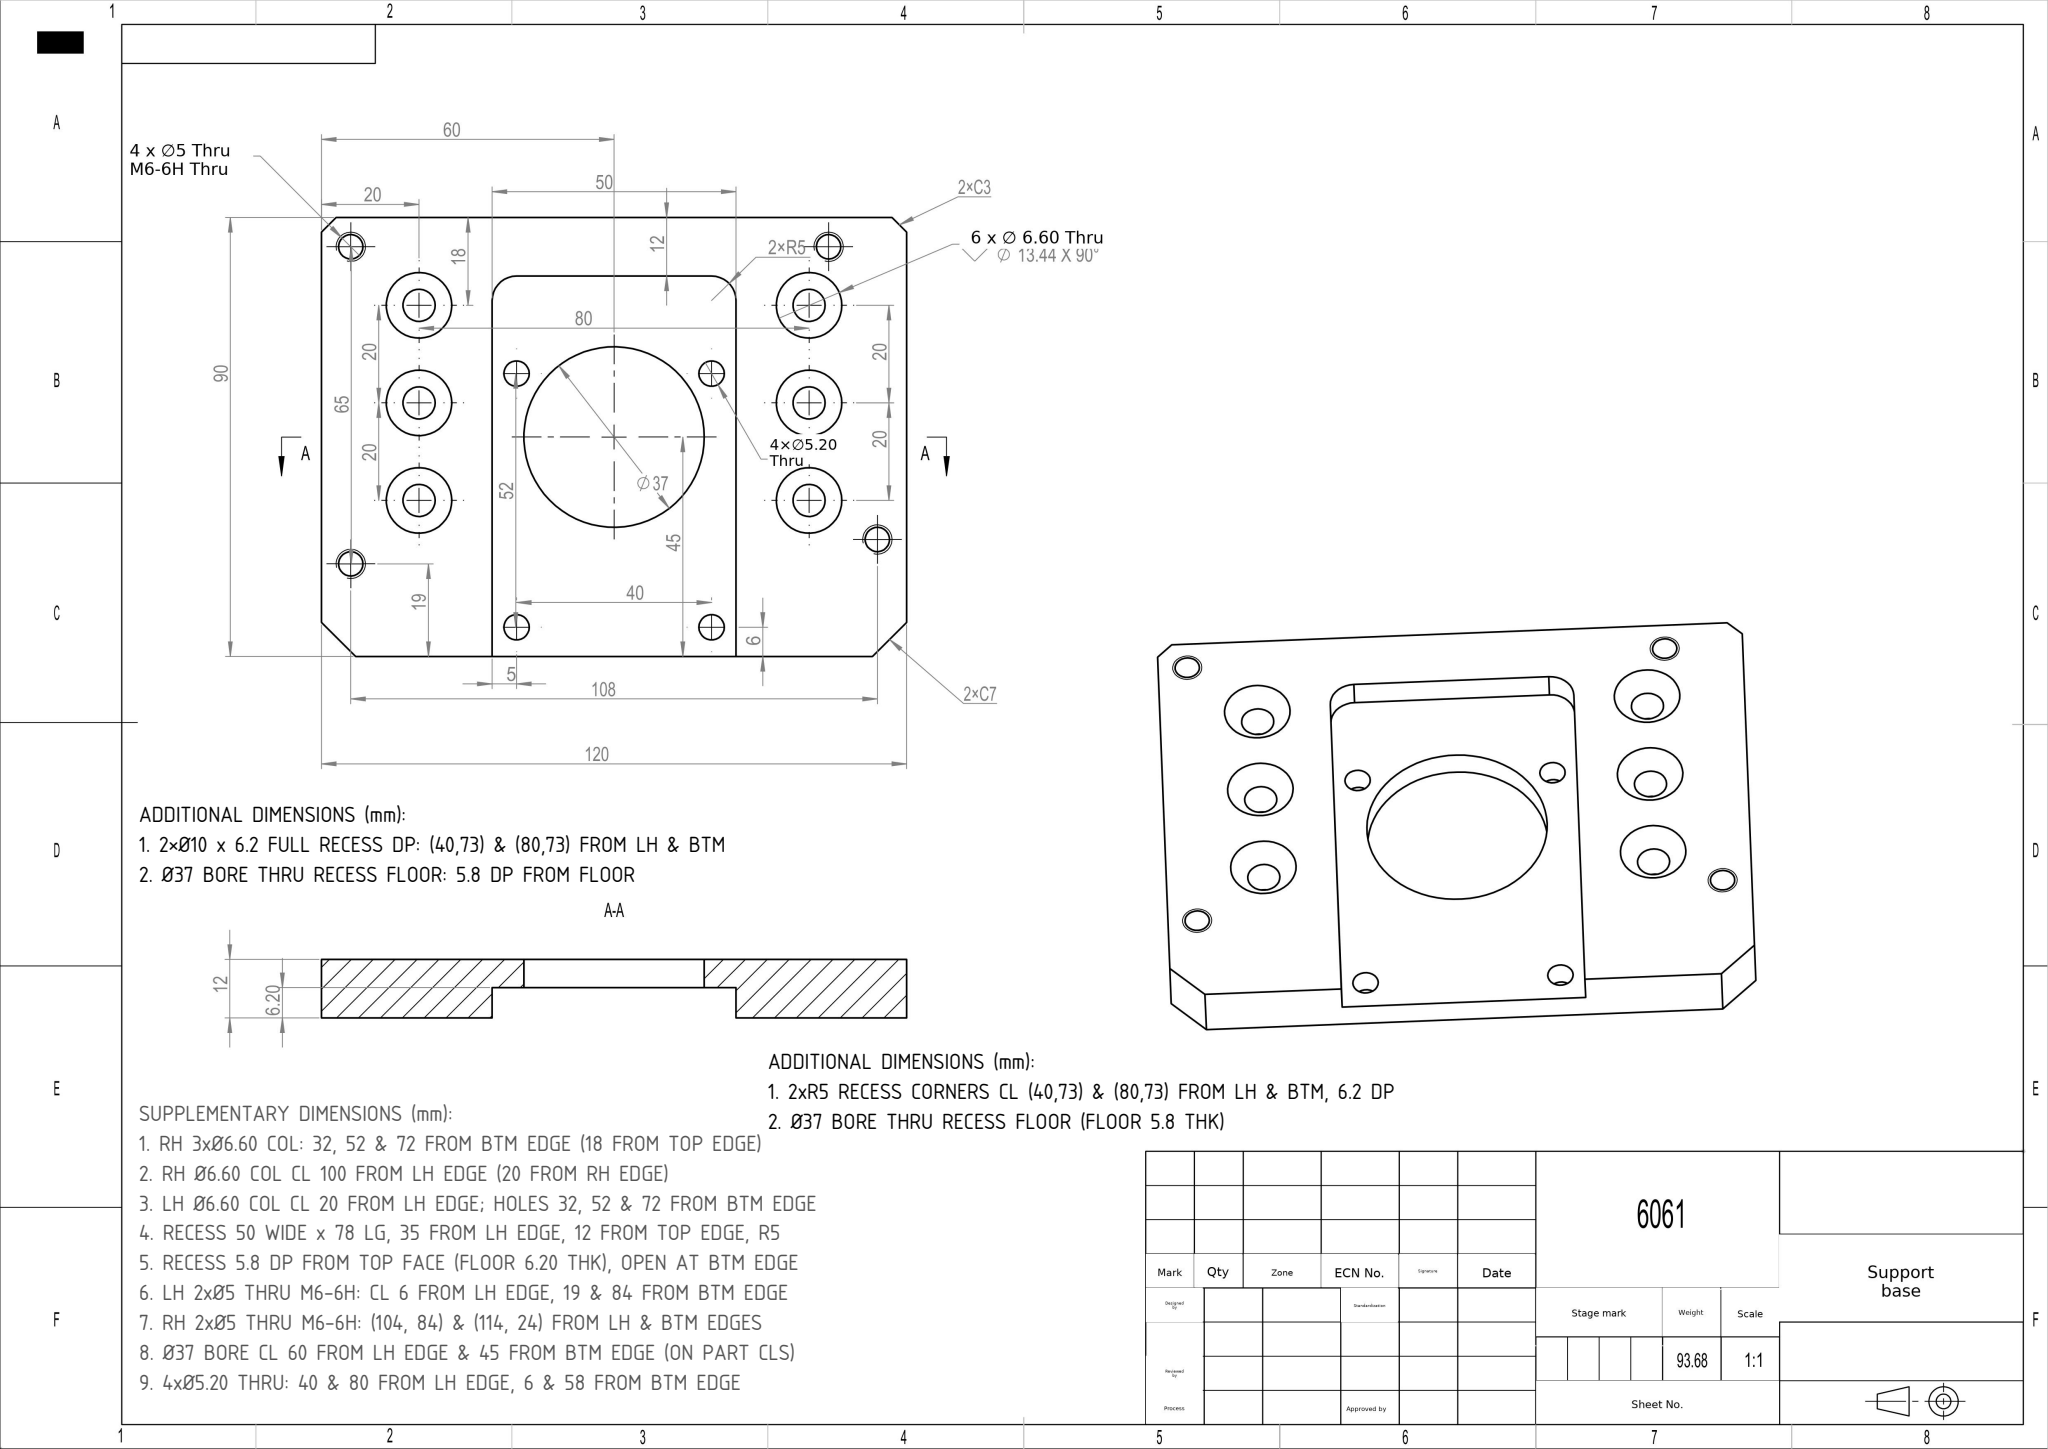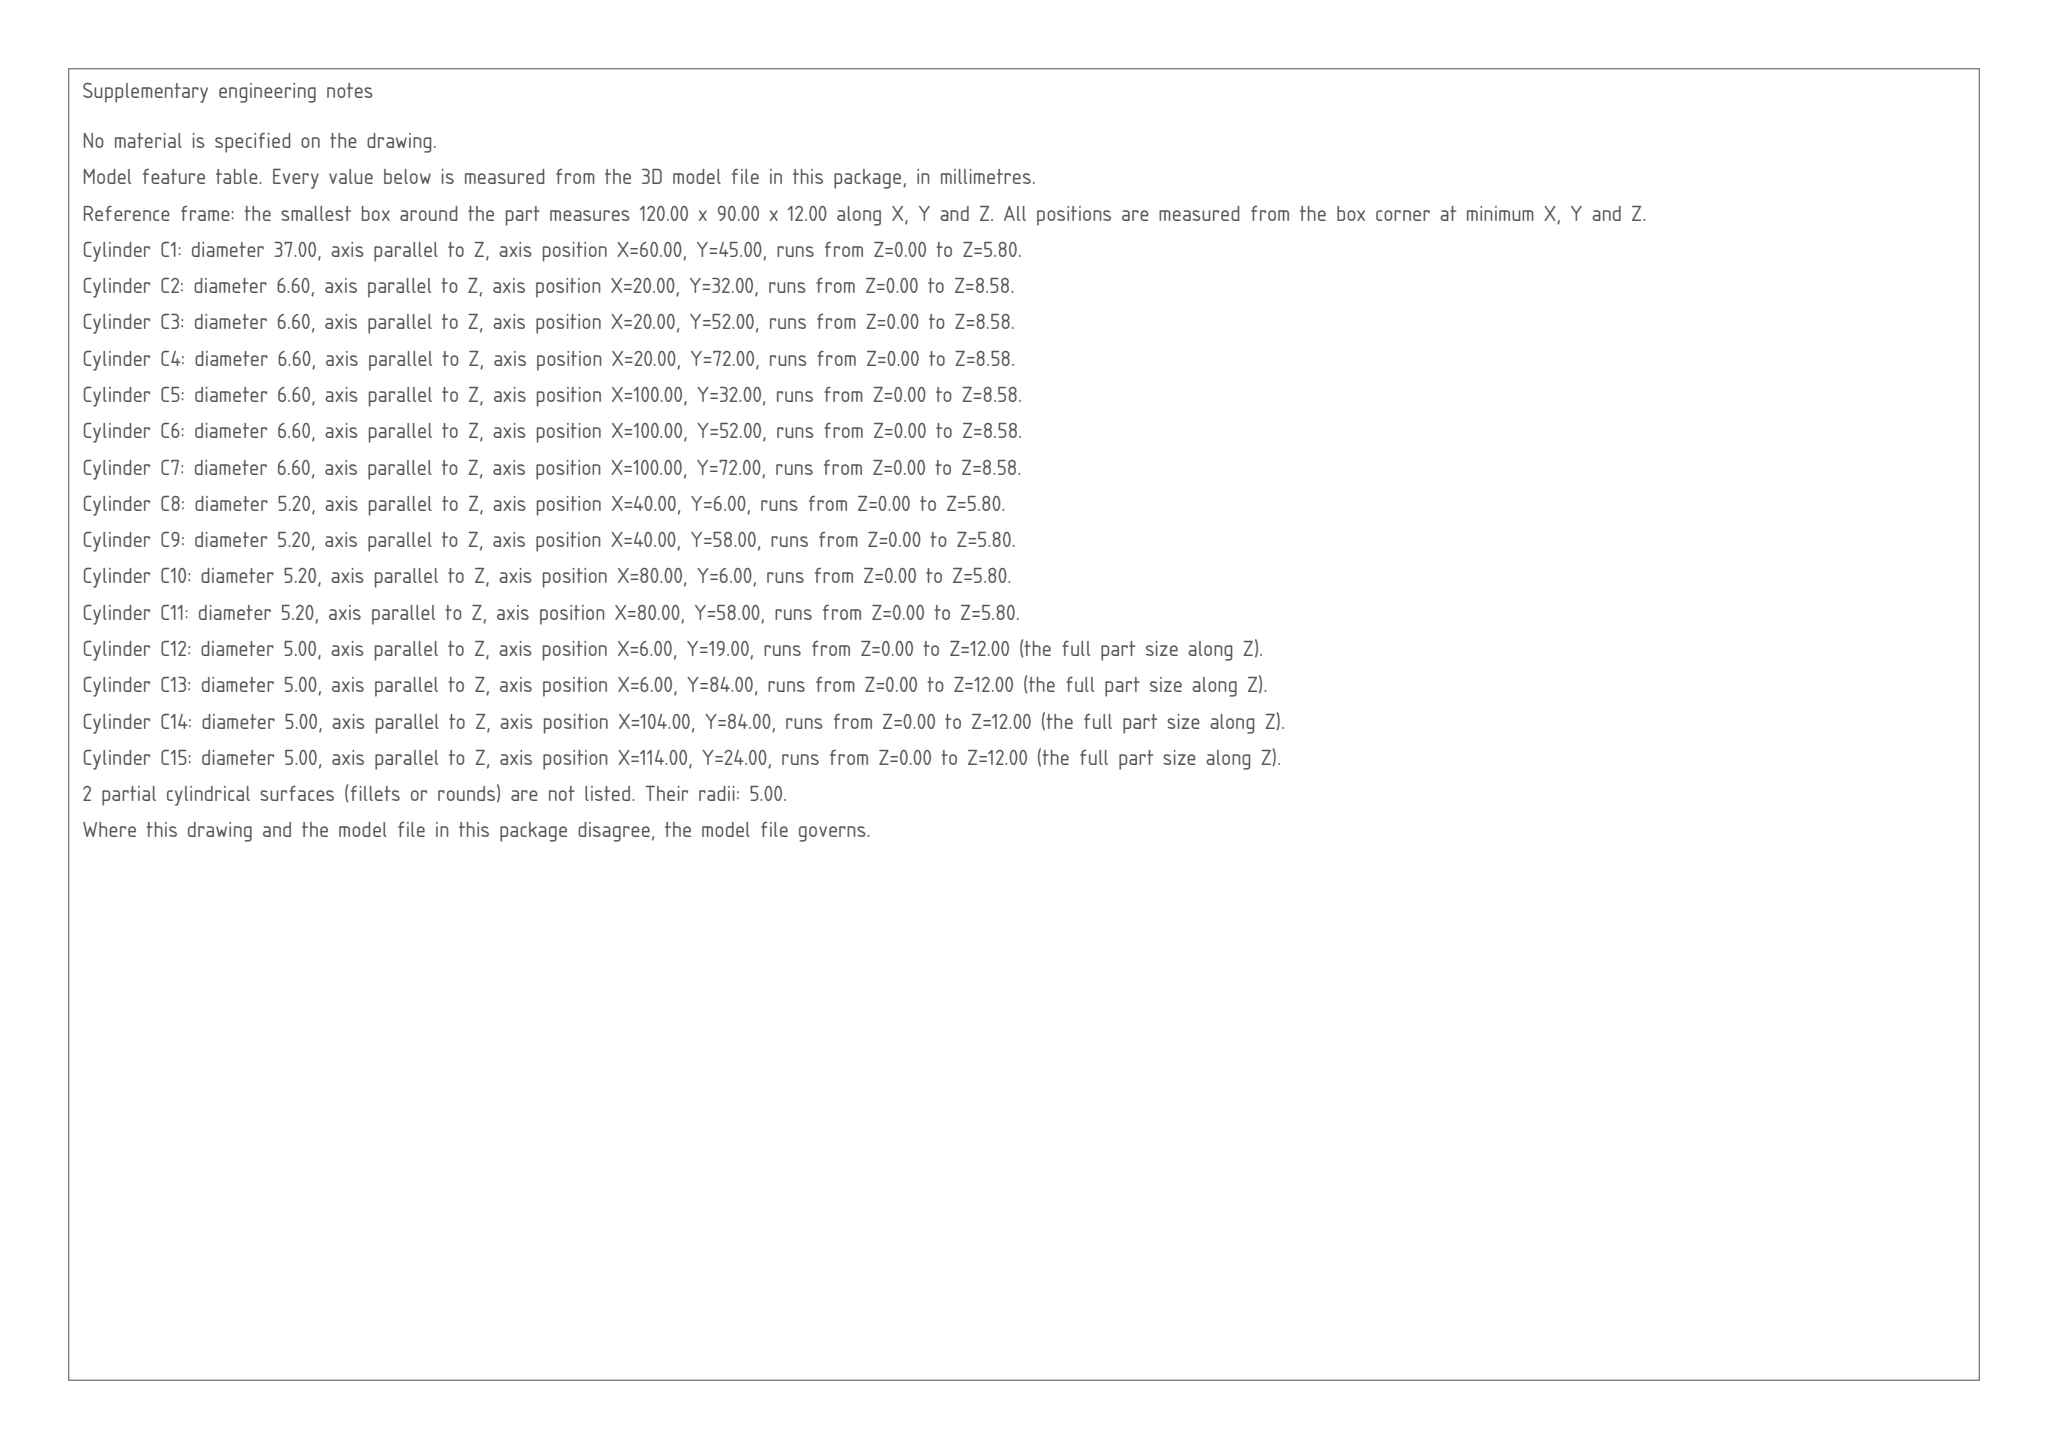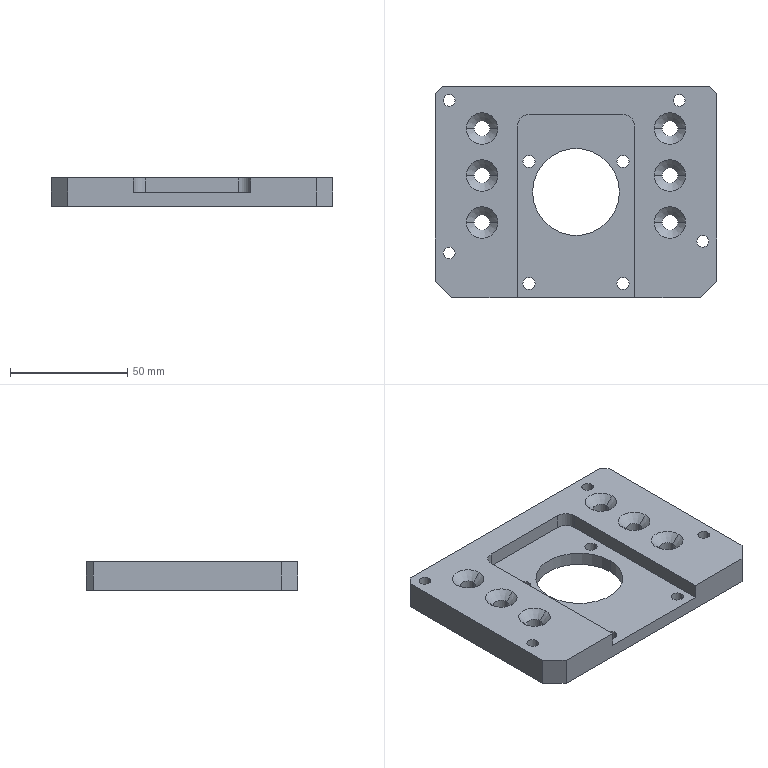Part | SolidWorks | mm | 1 solid | 58 faces | box 120 x 90 x 12 mm | volume 93677 mm3 | cylinder 32 | plane 14 | cone 12 | commonest cylinder face diameters 6.6 x12 5.2 x8 5 x8 37 x2 10 x2
build123d program:
from build123d import *

# Parameters (mm, degrees)
SKETCH1_W                                            = 120
SKETCH1_H                                            = 90
SKETCH1_R                                            = 18.5
BOSS_EXTRUDE1_DEPTH                                  = 12
M6_TAPPED_HOLE2_D                                    = 5
CHAMFER1_SIZE                                        = 3
CHAMFER2_SIZE                                        = 7
CUT_EXTRUDE1_START                                   = -6.2
SKETCH5_W                                            = 50
SKETCH5_H                                            = 78
SKETCH5_R                                            = 2.6
SKETCH5_R_2                                          = 18.5
CUT_EXTRUDE1_DEPTH                                   = 6.2
SKETCH6_R                                            = 2.6
CUT_EXTRUDE2_DEPTH                                   = 76.256
FILLET1_R                                            = 5
COUNTERSUNK_HOLE_FOR_M6_HEXAGON_SOCKET_C_D           = 6.6
COUNTERSUNK_HOLE_FOR_M6_HEXAGON_SOCKET_C_CSINK_D     = 13.44
COUNTERSUNK_HOLE_FOR_M6_HEXAGON_SOCKET_C_CSINK_ANGLE = 90
LPATTERN1_COUNT                                      = 3
LPATTERN1_PITCH                                      = 20
LPATTERN1_COUNT_DIR2                                 = 2
LPATTERN1_PITCH_DIR2                                 = 80


with BuildPart() as part:
    # Sketch1 → Boss-Extrude1 (new body)
    with BuildSketch(Plane.XY):
        Rectangle(SKETCH1_W, SKETCH1_H)
        Circle(SKETCH1_R, mode=Mode.SUBTRACT)
    extrude(amount=BOSS_EXTRUDE1_DEPTH)

    # M6 Tapped Hole2 (through all)
    with Locations(Plane.XY.offset(12)):
        with Locations((-54, 39), (44, 39), (54, -21), (-54, -26)):
            Hole(M6_TAPPED_HOLE2_D / 2)

    # Chamfer1
    chamfer1_edges = [part.edges().sort_by_distance(p)[0] for p in [
        (-60, 45, 6),
        (60, 45, 6),
    ]]
    chamfer(chamfer1_edges, length=CHAMFER1_SIZE)

    # Chamfer2
    chamfer2_edges = [part.edges().sort_by_distance(p)[0] for p in [
        (60, -45, 6),
        (-60, -45, 6),
    ]]
    chamfer(chamfer2_edges, length=CHAMFER2_SIZE)

    # Sketch5 → Cut-Extrude1 (cut)
    # profile 1 of 5: a face of its own
    with BuildSketch(Plane.XY.offset(12).offset(CUT_EXTRUDE1_START)):
        with Locations((0, -6)):
            Rectangle(SKETCH5_W, SKETCH5_H)
        with Locations((-20, -39)):
            Circle(SKETCH5_R, mode=Mode.SUBTRACT)
        with Locations((20, -39)):
            Circle(SKETCH5_R, mode=Mode.SUBTRACT)
        with Locations((-20, 13)):
            Circle(SKETCH5_R, mode=Mode.SUBTRACT)
        Circle(SKETCH5_R_2, mode=Mode.SUBTRACT)
        with Locations((20, 13)):
            Circle(SKETCH5_R, mode=Mode.SUBTRACT)
    # profile 2 of 5: a face of its own
    with BuildSketch(Plane.XY.offset(12).offset(CUT_EXTRUDE1_START)):
        with Locations((-20, 13)):
            Circle(SKETCH5_R)
    # profile 3 of 5: a face of its own
    with BuildSketch(Plane.XY.offset(12).offset(CUT_EXTRUDE1_START)):
        with Locations((20, 13)):
            Circle(SKETCH5_R)
    # profile 4 of 5: a face of its own
    with BuildSketch(Plane.XY.offset(12).offset(CUT_EXTRUDE1_START)):
        with Locations((20, -39)):
            Circle(SKETCH5_R)
    # profile 5 of 5: a face of its own
    with BuildSketch(Plane.XY.offset(12).offset(CUT_EXTRUDE1_START)):
        with Locations((-20, -39)):
            Circle(SKETCH5_R)
    extrude(amount=CUT_EXTRUDE1_DEPTH, mode=Mode.SUBTRACT)

    # Sketch6 → Cut-Extrude2 (cut, through all)
    with BuildSketch(Plane.XY.offset(5.8)):
        with Locations((20, 13)):
            Circle(SKETCH6_R)
        with Locations((20, -39)):
            Circle(SKETCH6_R)
        with Locations((-20, -39)):
            Circle(SKETCH6_R)
        with Locations((-20, 13)):
            Circle(SKETCH6_R)
    extrude(amount=-CUT_EXTRUDE2_DEPTH, mode=Mode.SUBTRACT)

    # Fillet1
    fillet1_edges = [part.edges().sort_by_distance(p)[0] for p in [
        (25, 33, 8.9),
        (-25, 33, 8.9),
    ]]
    fillet(fillet1_edges, radius=FILLET1_R)

    # Countersunk Hole for M6 Hexagon Socket C (through all)
    with Locations(Plane.XY.offset(12)):
        with Locations((-40, 27)):
            countersunk_hole_for_m6_hexagon_socket_c = CounterSinkHole(COUNTERSUNK_HOLE_FOR_M6_HEXAGON_SOCKET_C_D / 2, COUNTERSUNK_HOLE_FOR_M6_HEXAGON_SOCKET_C_CSINK_D / 2, counter_sink_angle=COUNTERSUNK_HOLE_FOR_M6_HEXAGON_SOCKET_C_CSINK_ANGLE)

    # LPattern1: Countersunk Hole for M6 Hexagon Socket C 3 × 2
    with Locations(*[(j * LPATTERN1_PITCH_DIR2, -i * LPATTERN1_PITCH, 0) for i in range(LPATTERN1_COUNT) for j in range(LPATTERN1_COUNT_DIR2) if (i, j) != (0, 0)]):
        add(countersunk_hole_for_m6_hexagon_socket_c, mode=Mode.SUBTRACT)


solid = part.part